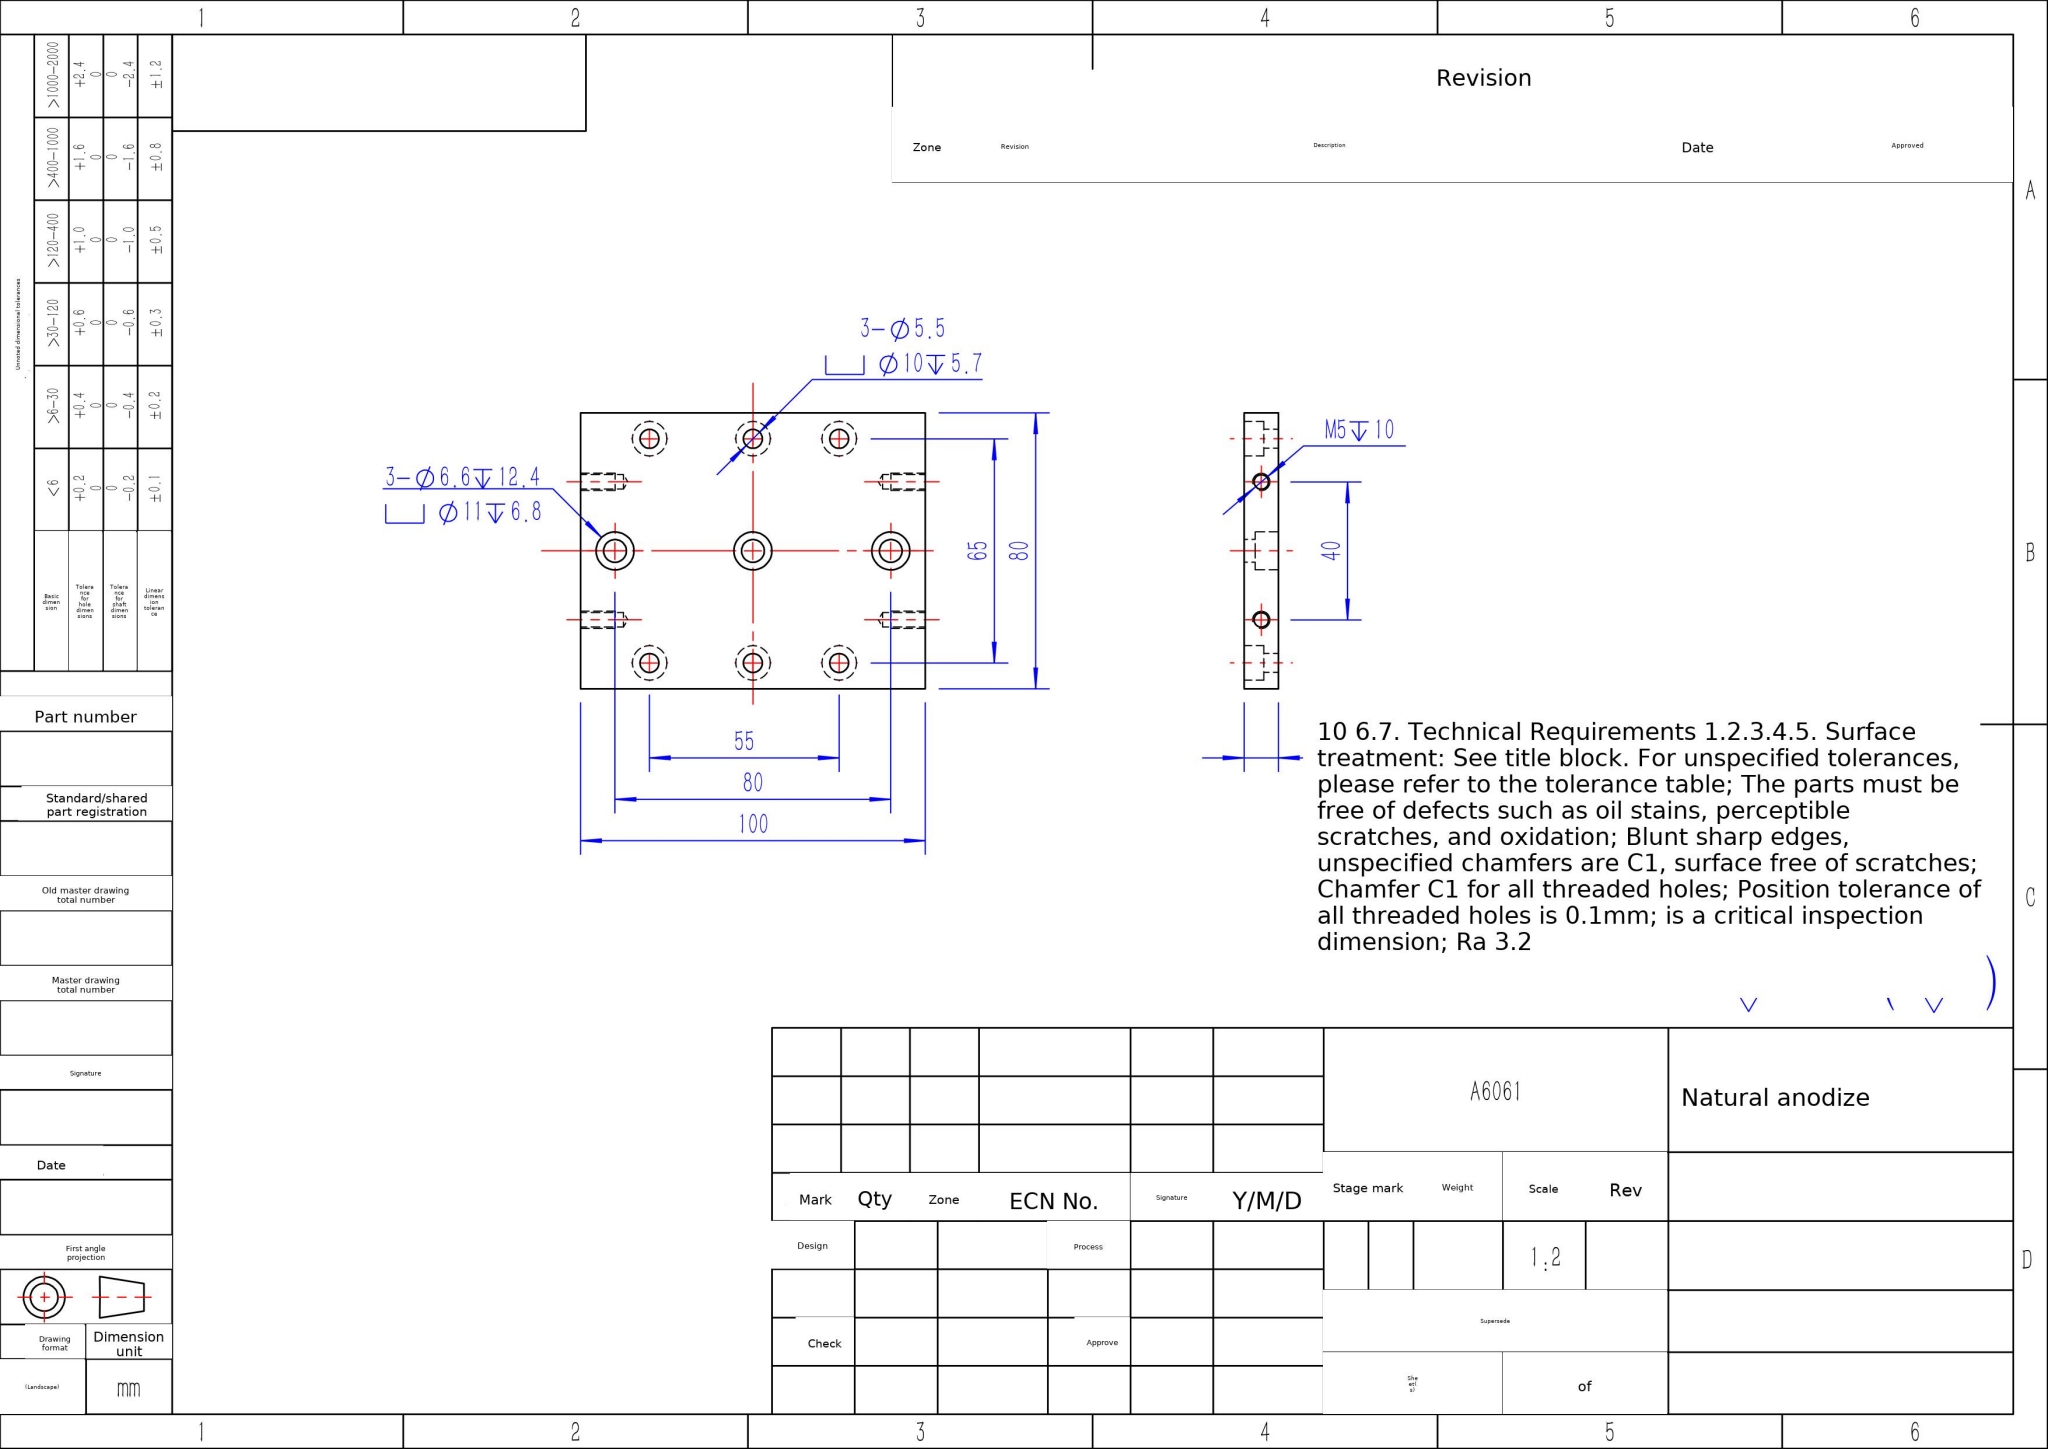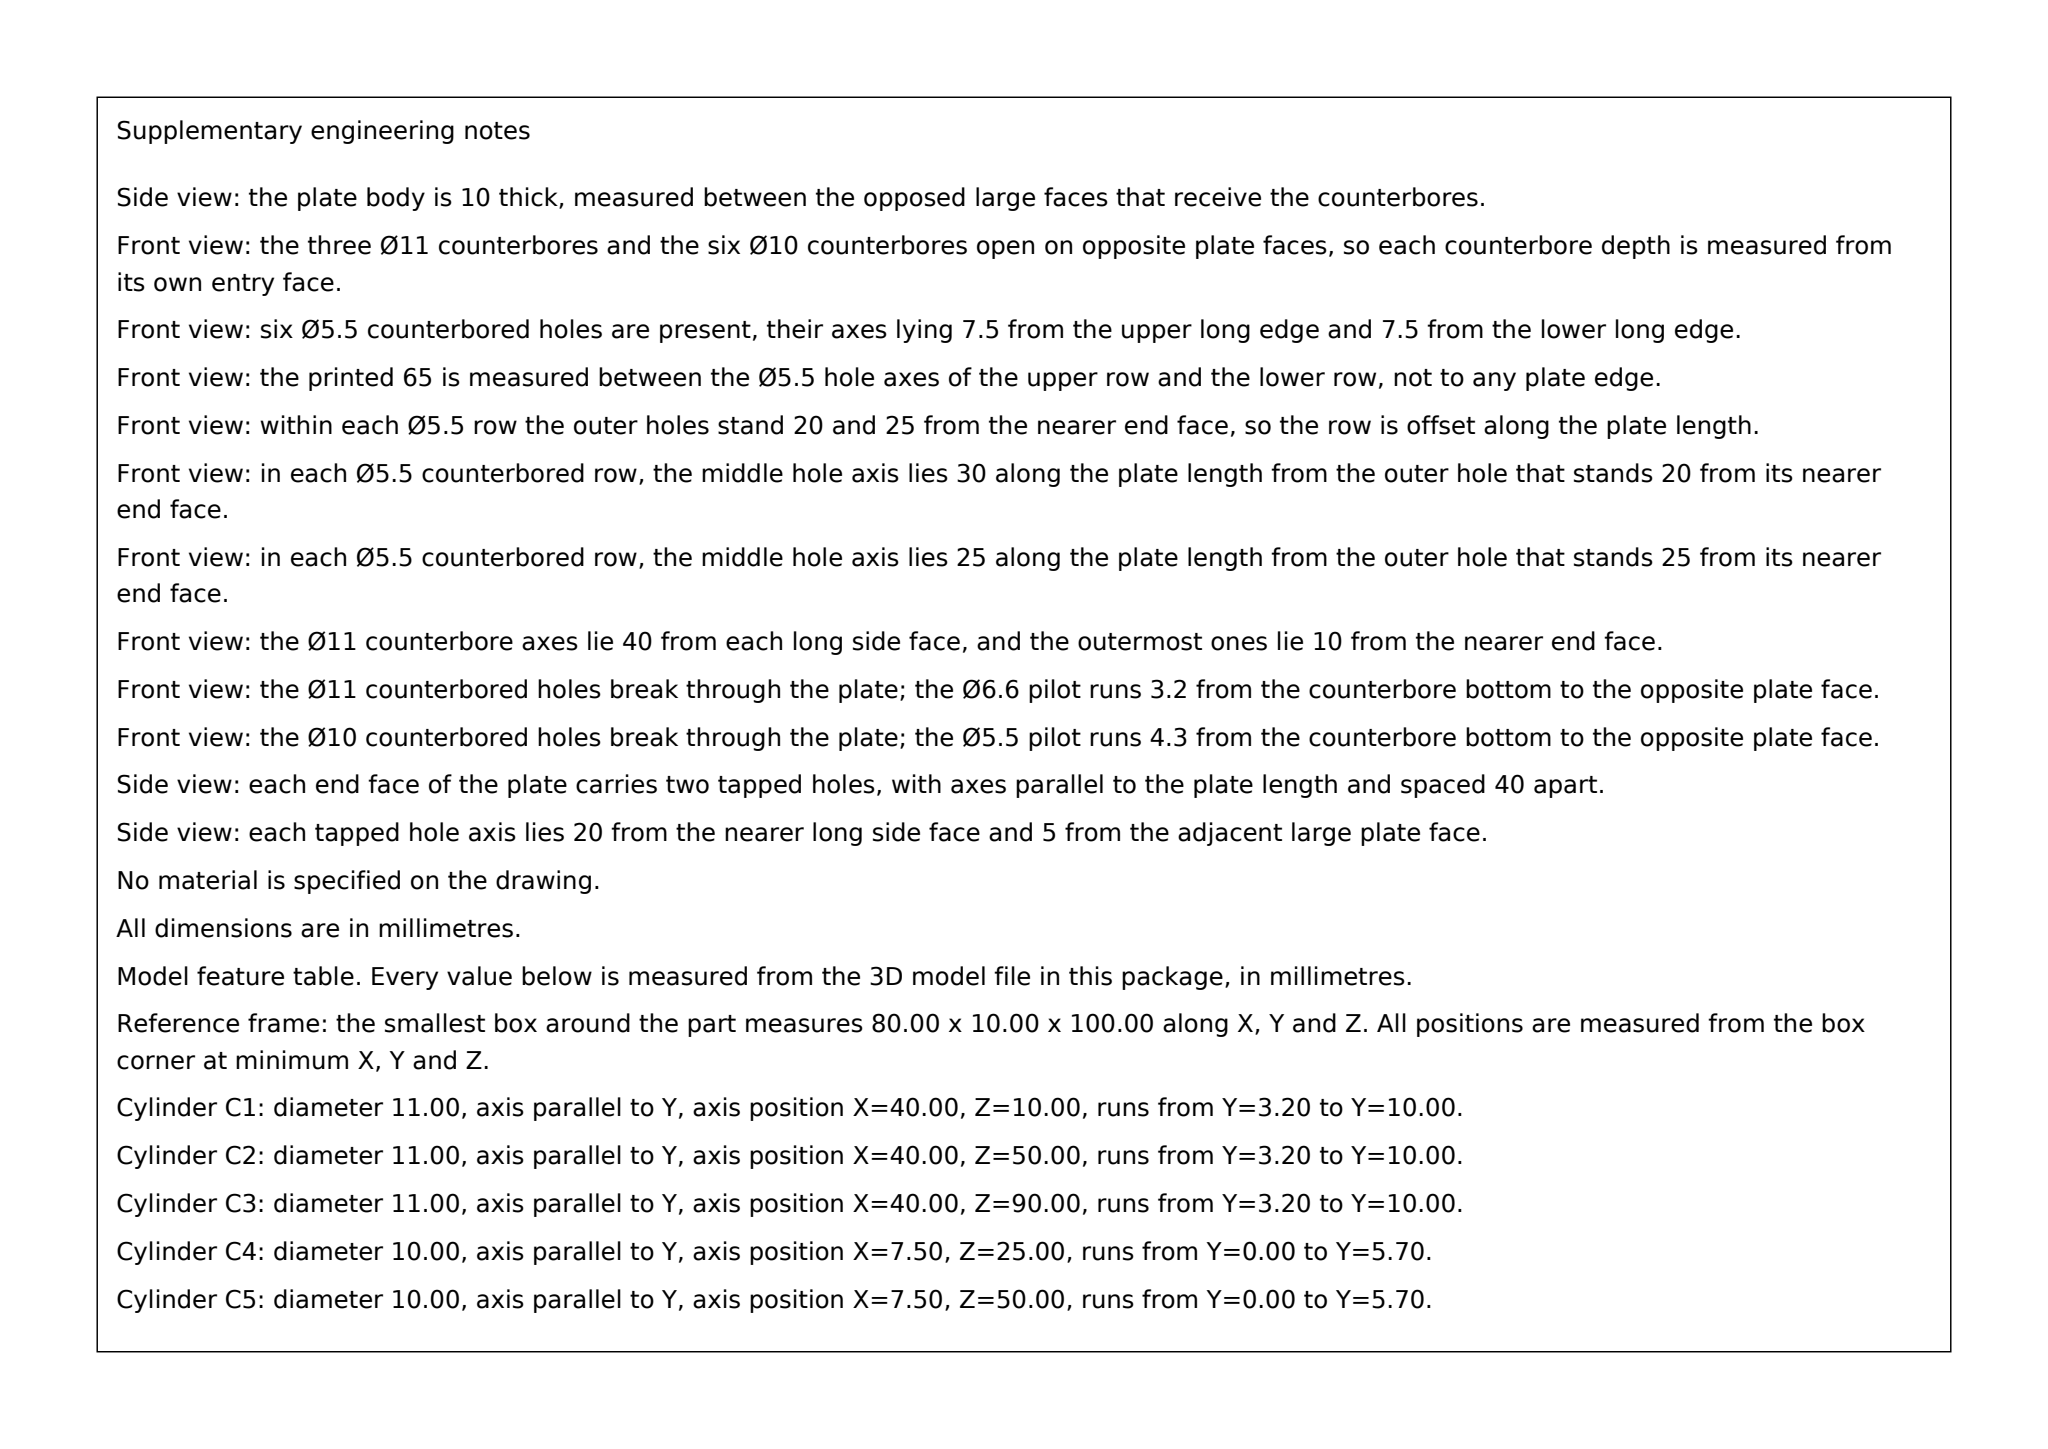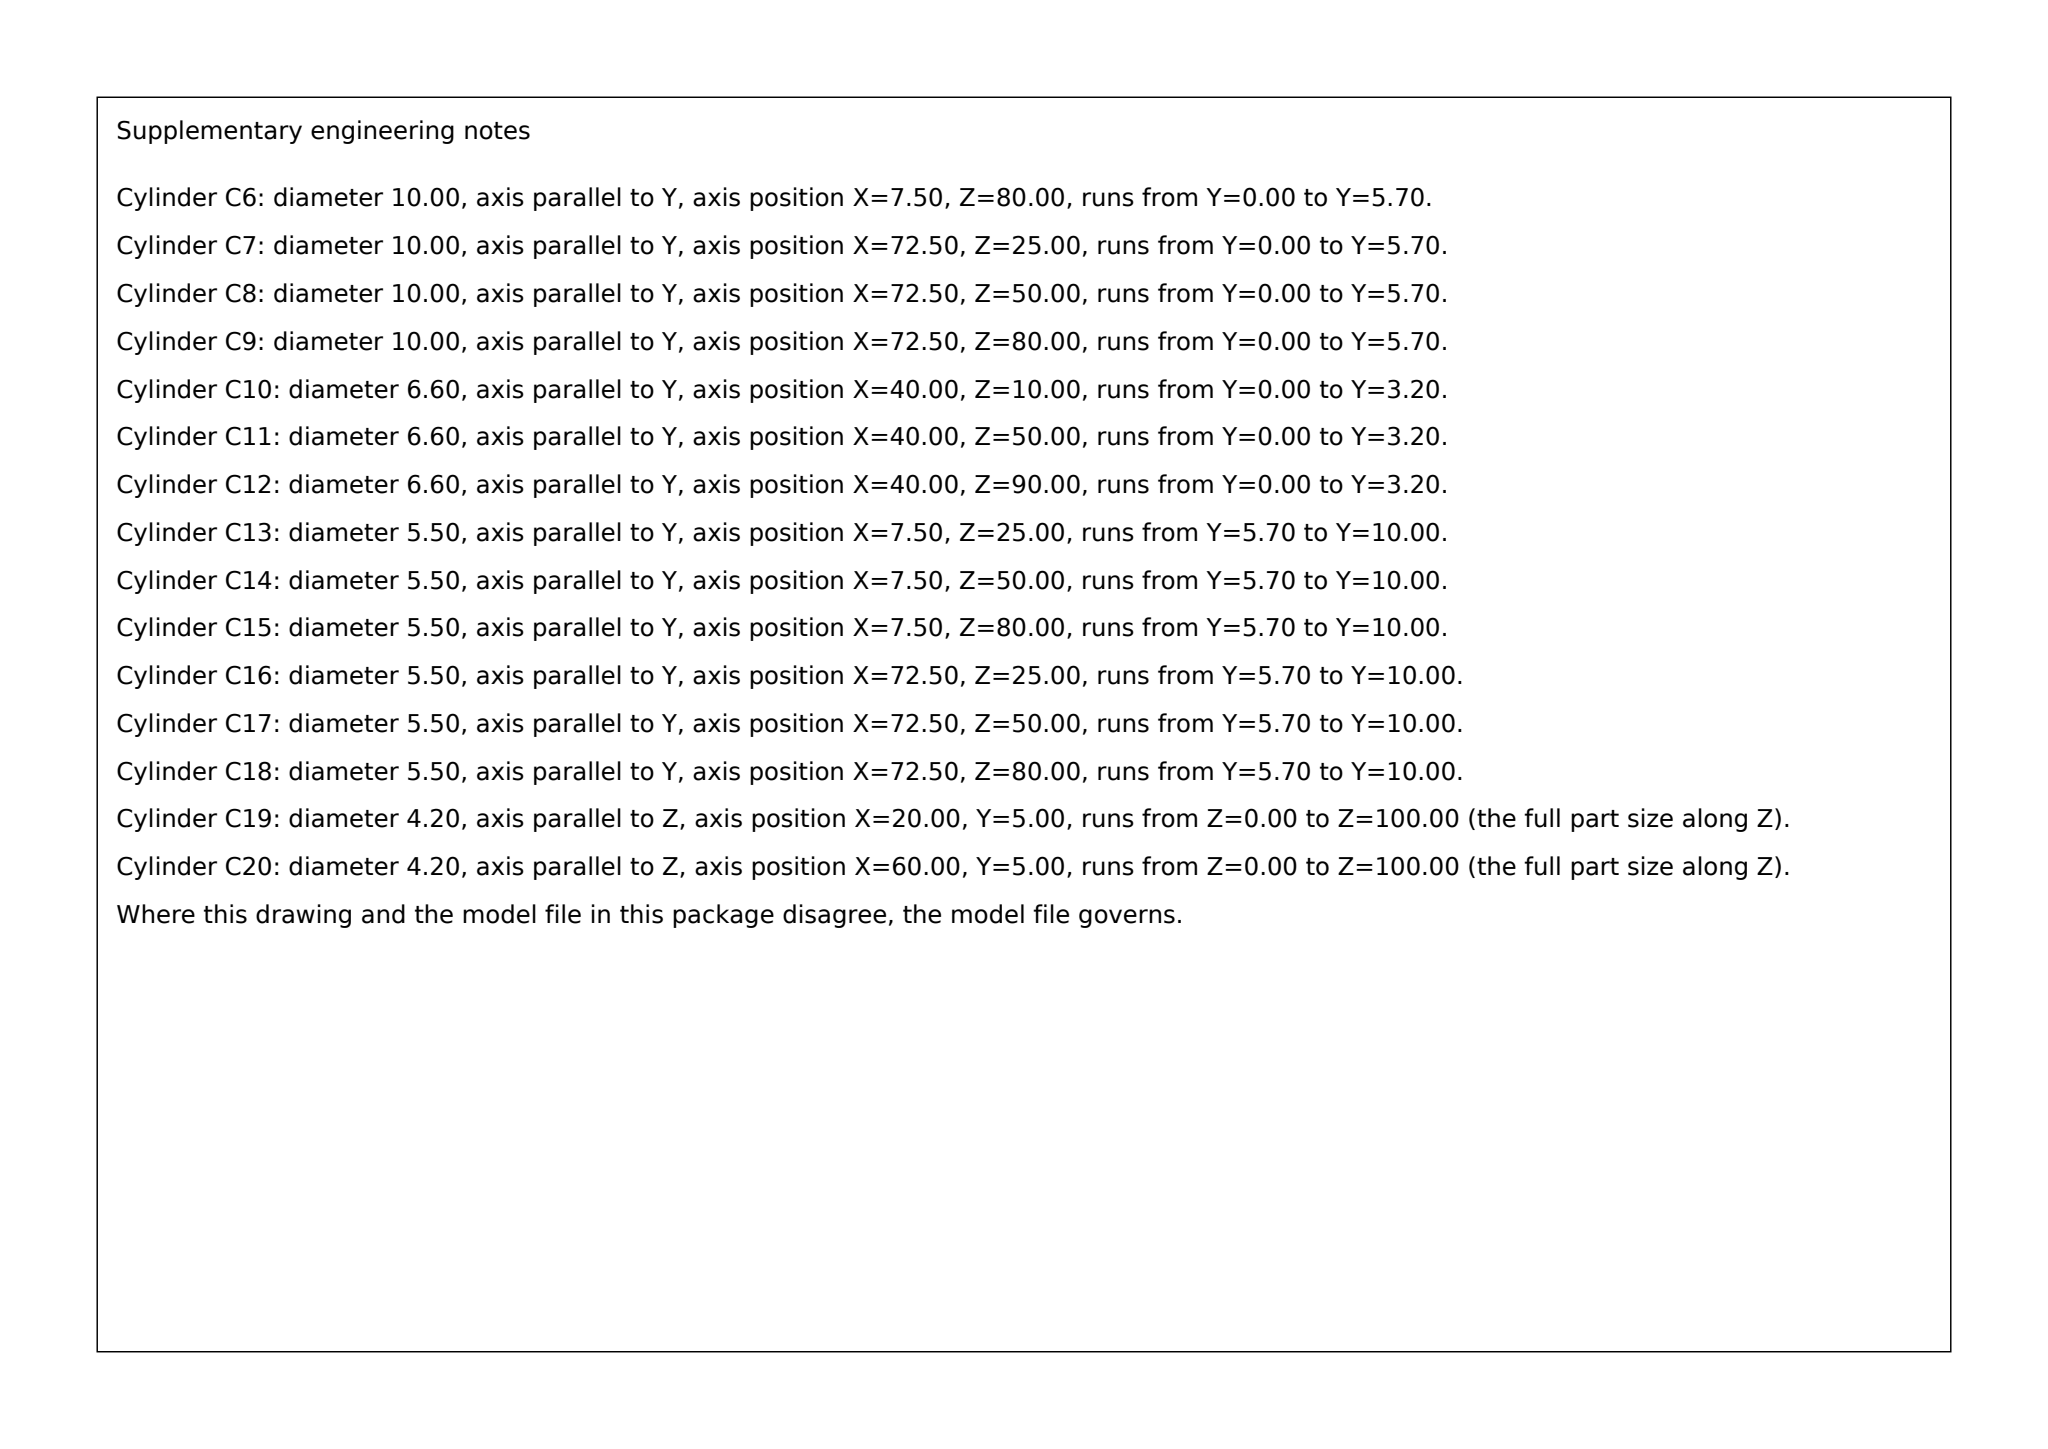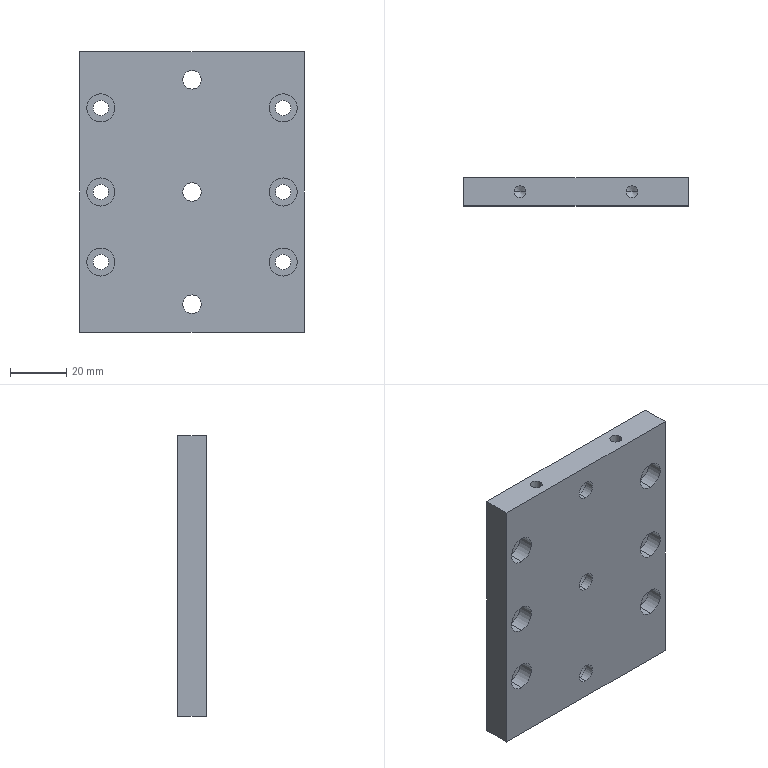Part | SolidWorks | mm | 1 solid | 67 faces | box 80 x 10 x 100 mm | volume 73723 mm3 | cylinder 44 | plane 15 | cone 8 | commonest cylinder face diameters 10 x12 5.5 x12 4.2 x8 11 x6 6.6 x6
Drawing notes:
PLATE 100 x 80 x 10 THK; 10 mm thickness measured between face A (counterbore face for Ø10) and face B (opposite). | from the solid: bbox_xyz [80,10,100]; axis_planes y=0.0 and y=10.0
6X Ø5.5 THRU, CBORE Ø10 DP 5.7 FROM FACE A; holes 7.5 from each 100 mm long edge; 25, 50 and 80 from the same 80 mm end face. | from the solid: cylinders Ø5.5 axis y at x=7.5 & 72.5, z=25/50/80, len 4.3; Ø10 axis y same positions, len 5.7; plane y=5.7
3X Ø6.6 THRU, CBORE Ø11 DP 6.8 FROM FACE B (face opposite the Ø10 counterbores); on 40 mm centreline from the 100 mm long edge; 10, 50 and 90 from the same 80 mm end face. | from the solid: cylinders Ø6.6 axis y at x=40, z=10/50/90, len 3.2; Ø11 axis y same positions, len 6.8; plane y=3.2
Ø6.6 portion is 3.2 deep from face A; remaining 6.8 is the Ø11 counterbore from face B (3.2 + 6.8 = 10 THRU). | from the solid: Ø6.6 len 3.2 + Ø11 len 6.8 = bbox y 10.0
4X M5 DP 10 (2 per end) in the two 80 x 10 end faces, at 20 and 60 from the 100 mm long edge, on mid-thickness 5 from face A. | from the solid: cylinders Ø4.2 axis z at (x=20,y=5) and (x=60,y=5), len 12.4; cones 118° ref_dia 4.2
build123d program:
from build123d import *

# Parameters (mm, degrees)
SKETCH1_W                                         = 80
SKETCH1_H                                         = 100
BOSS_EXTRUDE1_DEPTH                               = 10
M5_TAPPED_HOLE1_AT_2_COUNT                        = 2
M5_TAPPED_HOLE1_AT_2_PITCH                        = 40
HOLE_SIZE_ACCORDING_TO_HEXAGON_SOCKET_D           = 6.6
HOLE_SIZE_ACCORDING_TO_HEXAGON_SOCKET_DEPTH       = 12.4
HOLE_SIZE_ACCORDING_TO_HEXAGON_SOCKET_CBORE_D     = 11
HOLE_SIZE_ACCORDING_TO_HEXAGON_SOCKET_CBORE_DEPTH = 6.8
HOLE_SIZE_ACCORDING_TO_HEXAGON_SOCKET_TIP         = 1.983
HOLE_SIZE_ACCORDING_TO_HEXAGON_SO_2_D             = 5.5
HOLE_SIZE_ACCORDING_TO_HEXAGON_SO_2_DEPTH         = 12.4
HOLE_SIZE_ACCORDING_TO_HEXAGON_SO_2_CBORE_D       = 10
HOLE_SIZE_ACCORDING_TO_HEXAGON_SO_2_CBORE_DEPTH   = 5.7
HOLE_SIZE_ACCORDING_TO_HEXAGON_SO_2_TIP           = 1.652


with BuildPart() as part:
    # Sketch1 → Boss-Extrude1 (new body)
    with BuildSketch(Plane(origin=(0, 0, 0), x_dir=(1, 0, 0), z_dir=(0, 1, 0))):
        Rectangle(SKETCH1_W, SKETCH1_H)
    extrude(amount=BOSS_EXTRUDE1_DEPTH)

    # Sketch3 → M5 Tapped Hole1 (revolve, cut)
    with BuildSketch(Plane(origin=(-20, 5, 50), x_dir=(0, -1, 0), z_dir=(1, 0, 0))):
        Polygon((0, 0), (0, 13.662), (2.1, 12.4), (2.1, 0), align=None)
    m5_tapped_hole1 = revolve(axis=Axis((-20, 5, 56.35), (0, 0, -1)), mode=Mode.SUBTRACT)

    # M5 Tapped Hole1 at 2: M5 Tapped Hole1 ×2
    with Locations(*[(i * M5_TAPPED_HOLE1_AT_2_PITCH, 0, 0) for i in range(1, M5_TAPPED_HOLE1_AT_2_COUNT)]):
        add(m5_tapped_hole1, mode=Mode.SUBTRACT)

    # Mirror1: M5 Tapped Hole1 across plane
    add(m5_tapped_hole1.mirror(Plane.XY), mode=Mode.SUBTRACT)

    # Mirror1 copy 1 sketch → Mirror1 copy 1 (revolve, cut)
    with BuildSketch(Plane(origin=(20, 5, -50), x_dir=(0, -1, 0), z_dir=(1, 0, 0))):
        Polygon((0, 0), (0, -13.662), (2.1, -12.4), (2.1, 0), align=None)
    revolve(axis=Axis((20, 5, -56.35), (0, 0, -1)), mode=Mode.SUBTRACT)

    # Hole Size _ according to_ Hexagon Socket
    with Locations(Plane(origin=(0, 10, 0), x_dir=(1, 0, 0), z_dir=(0, 1, 0))):
        with Locations((0, -40), (0, 0), (0, 40)):
            CounterBoreHole(HOLE_SIZE_ACCORDING_TO_HEXAGON_SOCKET_D / 2, HOLE_SIZE_ACCORDING_TO_HEXAGON_SOCKET_CBORE_D / 2, HOLE_SIZE_ACCORDING_TO_HEXAGON_SOCKET_CBORE_DEPTH, depth=HOLE_SIZE_ACCORDING_TO_HEXAGON_SOCKET_DEPTH)
            with Locations((0, 0, -(HOLE_SIZE_ACCORDING_TO_HEXAGON_SOCKET_DEPTH + HOLE_SIZE_ACCORDING_TO_HEXAGON_SOCKET_TIP / 2))):  # 118° drill point
                Cone(0, HOLE_SIZE_ACCORDING_TO_HEXAGON_SOCKET_D / 2, HOLE_SIZE_ACCORDING_TO_HEXAGON_SOCKET_TIP, mode=Mode.SUBTRACT)

    # Hole Size _ according to_ Hexagon So 2
    with Locations(Plane(origin=(0, 0, 0), x_dir=(-1, 0, 0), z_dir=(0, -1, 0))):
        with Locations((-32.5, -30), (-32.5, 0), (-32.5, 25), (32.5, 25), (32.5, 0), (32.5, -30)):
            CounterBoreHole(HOLE_SIZE_ACCORDING_TO_HEXAGON_SO_2_D / 2, HOLE_SIZE_ACCORDING_TO_HEXAGON_SO_2_CBORE_D / 2, HOLE_SIZE_ACCORDING_TO_HEXAGON_SO_2_CBORE_DEPTH, depth=HOLE_SIZE_ACCORDING_TO_HEXAGON_SO_2_DEPTH)
            with Locations((0, 0, -(HOLE_SIZE_ACCORDING_TO_HEXAGON_SO_2_DEPTH + HOLE_SIZE_ACCORDING_TO_HEXAGON_SO_2_TIP / 2))):  # 118° drill point
                Cone(0, HOLE_SIZE_ACCORDING_TO_HEXAGON_SO_2_D / 2, HOLE_SIZE_ACCORDING_TO_HEXAGON_SO_2_TIP, mode=Mode.SUBTRACT)


solid = part.part